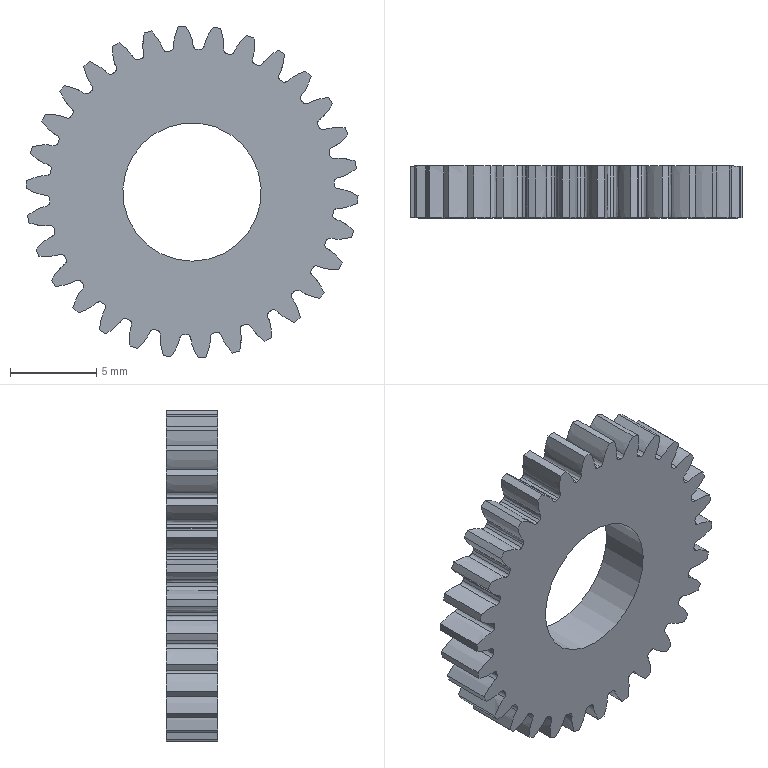Component | NX | 30_GEAR_2 | 1 solid | 183 faces | volume 605 mm3 | other 150 | cylinder 31 | plane 2 | commonest cylinder face diameters 16.5 x30 8 x1